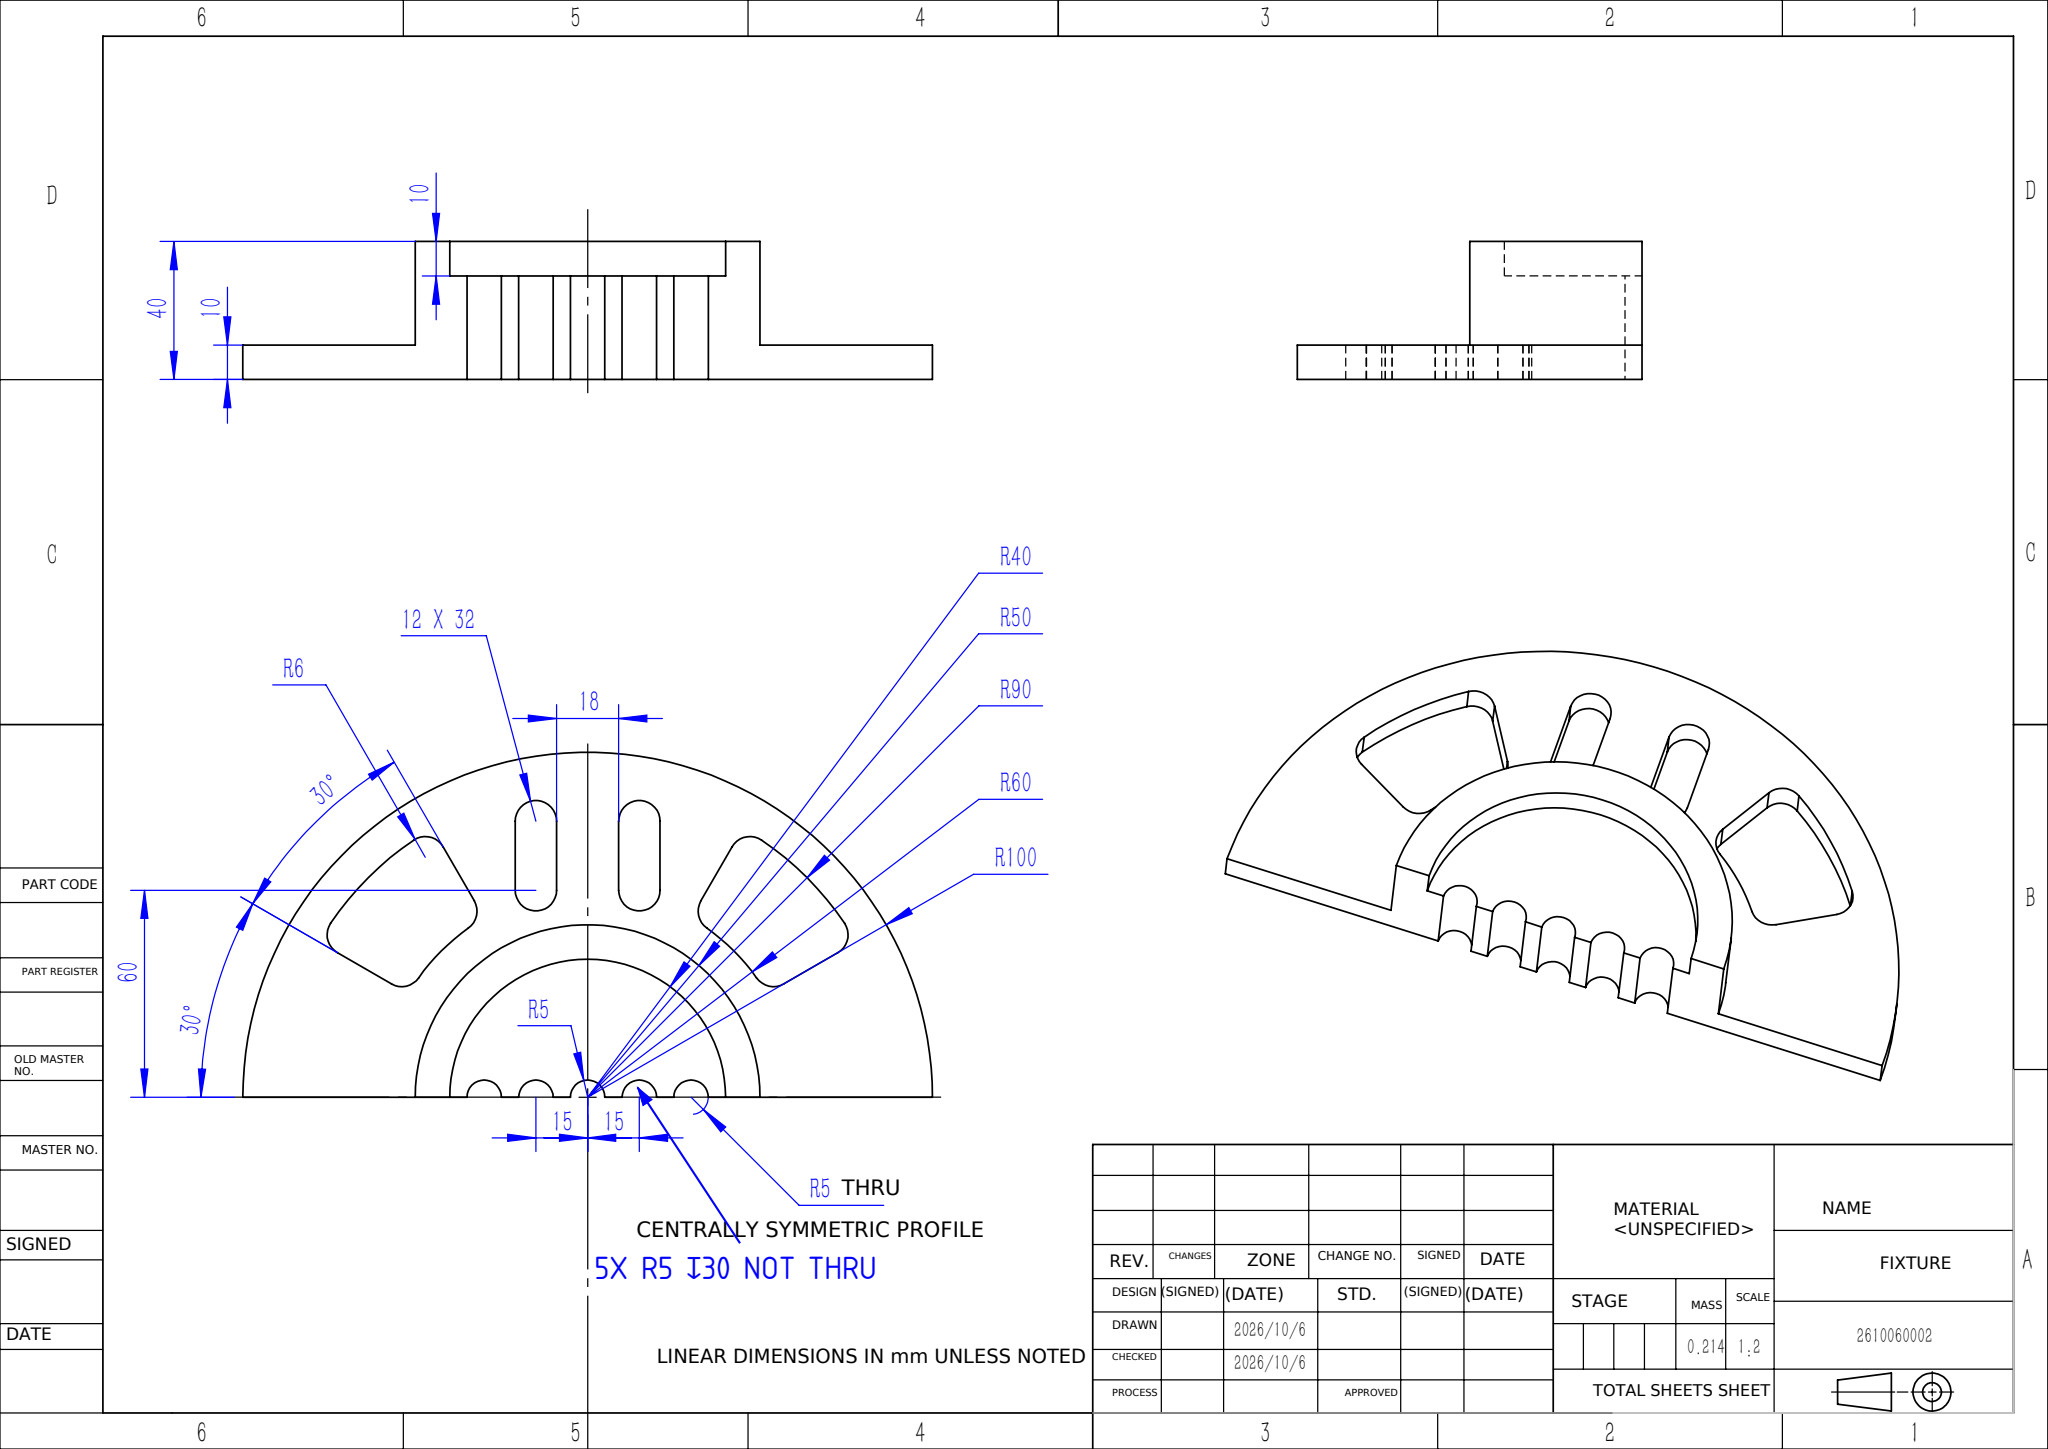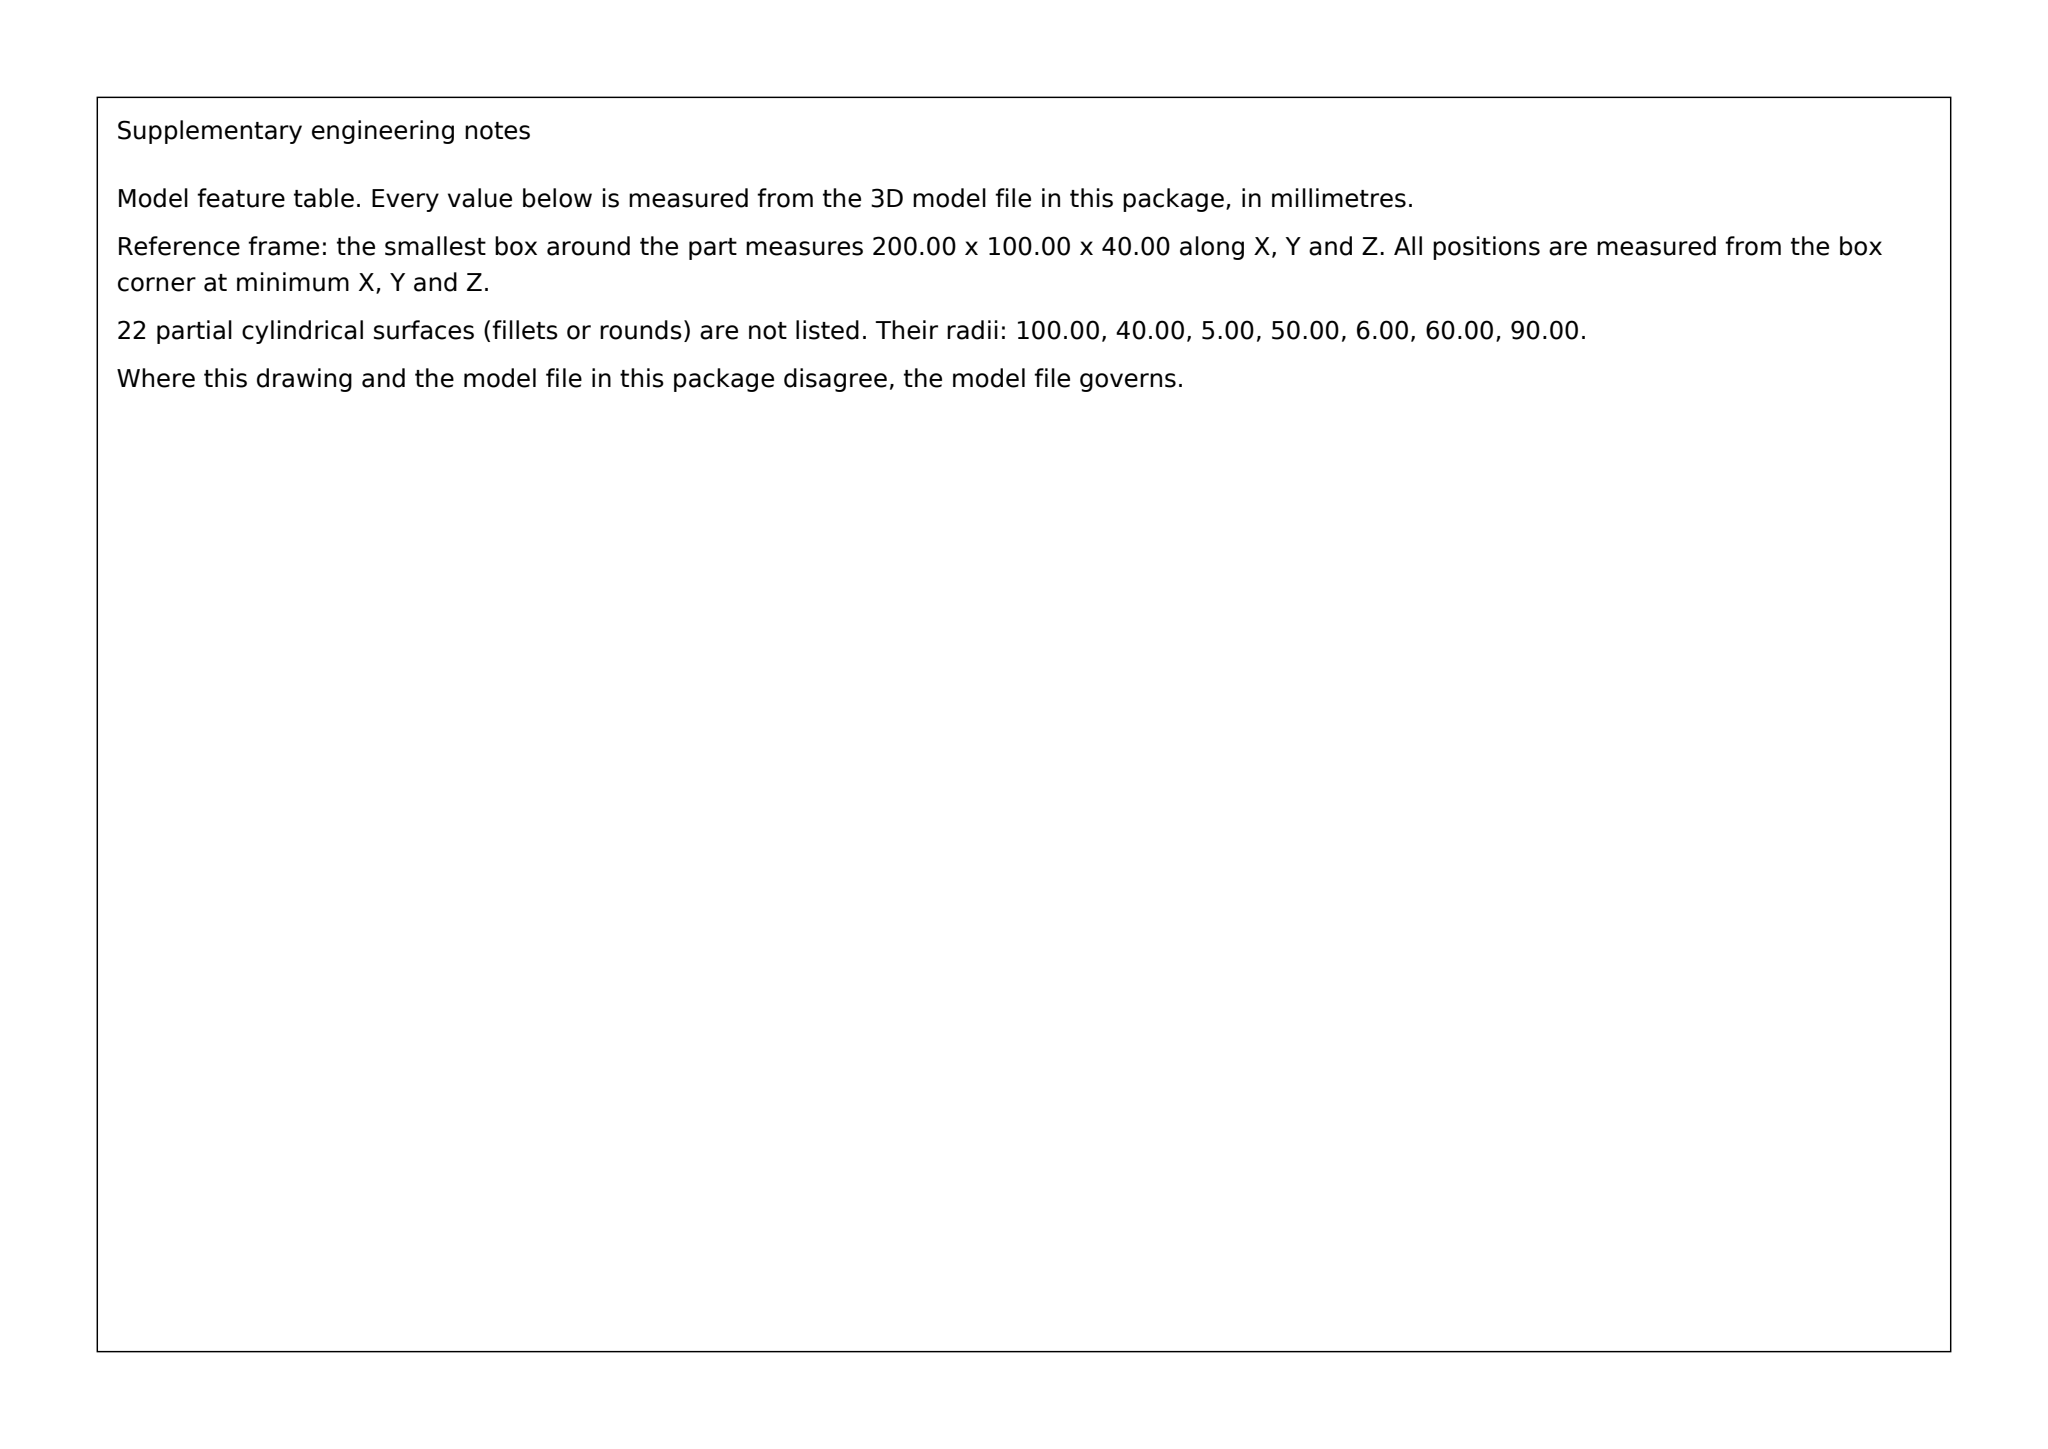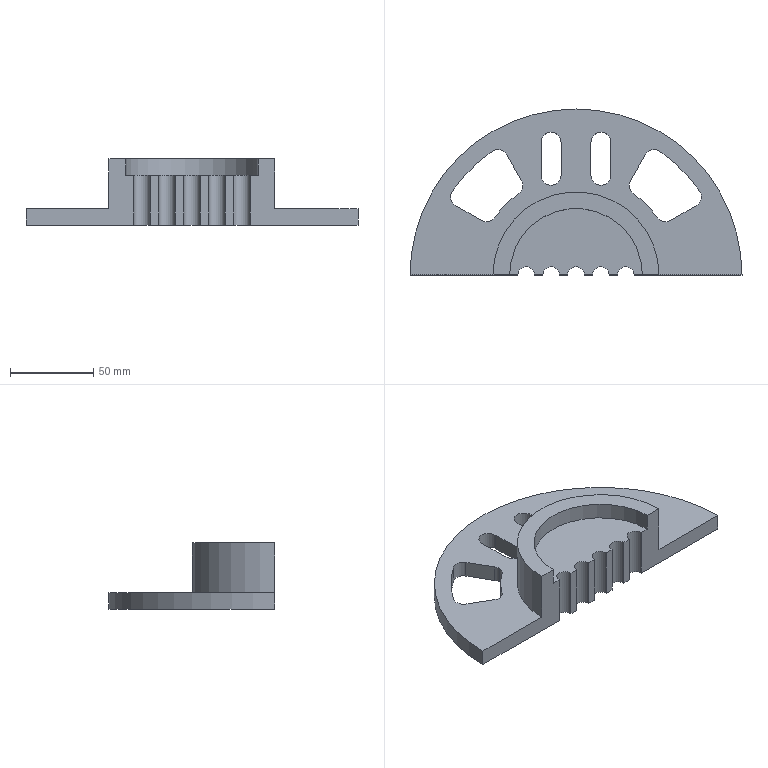Part | SolidWorks | mm | 1 solid | 44 faces | box 200 x 100 x 40 mm | volume 213854 mm3 | cylinder 26 | plane 18 | commonest cylinder face diameters 12 x14 10 x5 120 x2 180 x2 100 x1 200 x1 80 x1
Drawing notes:
5X R5 SCALLOP, DP 30 FROM BOTTOM FACE - NOT THRU | from the solid: Five Ø10 concave arcs (180 deg) on y=0 at x=70,85,100,115,130, z from 0 to 30; part height 40
build123d program:
from build123d import *

# Parameters (mm, degrees)
BOSS_EXTRUDE1_DEPTH = 30
BOSS_EXTRUDE2_DEPTH = 10
CUT_EXTRUDE1_DEPTH  = 145.568
CUT_EXTRUDE2_DEPTH  = 145.568
CUT_EXTRUDE3_DEPTH  = 10
CUT_EXTRUDE4_DEPTH  = 145.568


with BuildPart() as part:
    # Sketch1 → Boss-Extrude1 (new body)
    with BuildSketch(Plane.XY):
        with BuildLine():
            Line((-50, 0), (50, 0))
            ThreePointArc((50, 0), (0, 50), (-50, 0))
        make_face()
    extrude(amount=-BOSS_EXTRUDE1_DEPTH)

    # Sketch2 → Boss-Extrude2 (add)
    with BuildSketch(Plane(origin=(0, 0, -30), x_dir=(-1, 0, 0), z_dir=(0, 0, -1))):
        with BuildLine():
            Line((100, 0), (-100, 0))
            ThreePointArc((-100, 0), (0, 100), (100, 0))
        make_face()
    extrude(amount=BOSS_EXTRUDE2_DEPTH)

    # Sketch3 → Cut-Extrude1 (cut, through all)
    with BuildSketch(Plane.XY.offset(-30)):
        with BuildLine():
            Line((-72.56, 41.893), (-56.921, 32.863))
            ThreePointArc((-56.921, 32.863), (-52.633, 32.199), (-49.019, 34.6))
            ThreePointArc((-49.019, 34.6), (-42.426, 42.426), (-34.6, 49.019))
            ThreePointArc((-34.6, 49.019), (-32.199, 52.633), (-32.863, 56.921))
            Line((-32.863, 56.921), (-41.893, 72.56))
            ThreePointArc((-41.893, 72.56), (-45.744, 75.408), (-50.452, 74.529))
            ThreePointArc((-50.452, 74.529), (-63.64, 63.64), (-74.529, 50.452))
            ThreePointArc((-74.529, 50.452), (-75.408, 45.744), (-72.56, 41.893))
        make_face()
        with BuildLine():
            Line((41.893, 72.56), (32.863, 56.921))
            ThreePointArc((32.863, 56.921), (32.199, 52.633), (34.6, 49.019))
            ThreePointArc((34.6, 49.019), (42.426, 42.426), (49.019, 34.6))
            ThreePointArc((49.019, 34.6), (52.633, 32.199), (56.921, 32.863))
            Line((56.921, 32.863), (72.56, 41.893))
            ThreePointArc((72.56, 41.893), (75.408, 45.744), (74.529, 50.452))
            ThreePointArc((74.529, 50.452), (63.64, 63.64), (50.452, 74.529))
            ThreePointArc((50.452, 74.529), (45.744, 75.408), (41.893, 72.56))
        make_face()
    extrude(amount=-CUT_EXTRUDE1_DEPTH, mode=Mode.SUBTRACT)

    # Sketch4 → Cut-Extrude2 (cut, through all)
    with BuildSketch(Plane.XY.offset(-30)):
        with BuildLine():
            Line((-9, 80), (-9, 60))
            ThreePointArc((-9, 60), (-15, 54), (-21, 60))
            Line((-21, 60), (-21, 80))
            ThreePointArc((-21, 80), (-15, 86), (-9, 80))
        make_face()
        with BuildLine():
            Line((9, 80), (9, 60))
            ThreePointArc((9, 60), (15, 54), (21, 60))
            Line((21, 60), (21, 80))
            ThreePointArc((21, 80), (15, 86), (9, 80))
        make_face()
    extrude(amount=-CUT_EXTRUDE2_DEPTH, mode=Mode.SUBTRACT)

    # Sketch5 → Cut-Extrude3 (cut)
    with BuildSketch(Plane.XY):
        with BuildLine():
            Line((-40, 0), (40, 0))
            ThreePointArc((40, 0), (0, 40), (-40, 0))
        make_face()
    extrude(amount=-CUT_EXTRUDE3_DEPTH, mode=Mode.SUBTRACT)

    # Sketch6 → Cut-Extrude4 (cut, through all)
    with BuildSketch(Plane.XY.offset(-10)):
        with BuildLine():
            Line((-5, 0), (5, 0))
            ThreePointArc((5, 0), (0, 5), (-5, 0))
        make_face()
        with BuildLine():
            Line((-20, 0), (-10, 0))
            ThreePointArc((-10, 0), (-15, 5), (-20, 0))
        make_face()
        with BuildLine():
            Line((25, 0), (35, 0))
            ThreePointArc((35, 0), (30, 5), (25, 0))
        make_face()
        with BuildLine():
            Line((10, 0), (20, 0))
            ThreePointArc((20, 0), (15, 5), (10, 0))
        make_face()
        with BuildLine():
            Line((-35, 0), (-25, 0))
            ThreePointArc((-25, 0), (-30, 5), (-35, 0))
        make_face()
    extrude(amount=-CUT_EXTRUDE4_DEPTH, mode=Mode.SUBTRACT)


solid = part.part